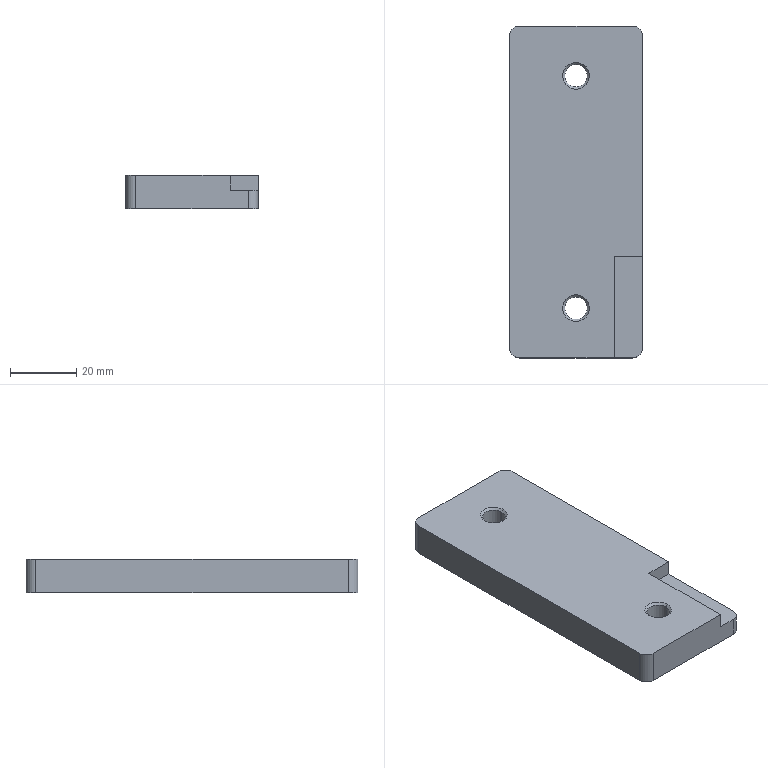Component | SolidWorks | FrameAssembly-1_FrameWeldment-1_MountingPlate-3 | 1 solid | 21 faces | box 40 x 100 x 10 mm | volume 38030 mm3 | plane 9 | cylinder 8 | cone 4 | commonest cylinder face diameters 6.8 x4 6 x4
build123d program:
from build123d import *

# Parameters (mm, degrees)
SKETCH1_2_W                = 40
SKETCH1_2_H                = 100
BOSS_EXTRUDE1_DEPTH        = 10
F_6_8_6_8_DIAMETER_HOLE1_D = 6.8
CHAMFER1_SIZE              = 0.625
FILLET1_R                  = 3
SKETCH1_W                  = 9
SKETCH1_H                  = 31
HOOK_CLEARANCE_SLOT_DEPTH  = 4.5


with BuildPart() as part:
    # Sketch1_2 → Boss-Extrude1 (new body)
    with BuildSketch(Plane.XY.offset(5)):
        Rectangle(SKETCH1_2_W, SKETCH1_2_H)
    extrude(amount=-BOSS_EXTRUDE1_DEPTH)

    # 6.8 _6.8_ Diameter Hole1 (through all)
    with Locations(Plane.XY.offset(5)):
        with Locations((0, -35), (0, 35)):
            Hole(F_6_8_6_8_DIAMETER_HOLE1_D / 2)

    # Chamfer1
    chamfer1_edges = [part.edges().sort_by_distance(p)[0] for p in [
        (3.4, 35, 5),
        (3.4, -35, 5),
    ]]
    chamfer(chamfer1_edges, length=CHAMFER1_SIZE)

    # Fillet1
    fillet1_edges = [part.edges().sort_by_distance(p)[0] for p in [
        (-20, -50, 0),
        (-20, 50, 0),
        (20, 50, 0),
        (20, -50, 0),
    ]]
    fillet(fillet1_edges, radius=FILLET1_R)

    # Sketch1 → Hook Clearance Slot (cut)
    with BuildSketch(Plane.XY.offset(5)):
        with Locations((16, -35)):
            Rectangle(SKETCH1_W, SKETCH1_H)
    extrude(amount=-HOOK_CLEARANCE_SLOT_DEPTH, mode=Mode.SUBTRACT)


solid = part.part

# Placed as in the assembly
solid = solid.moved(Location((43.754, -329.627, -371.5), (0, 0, 0)))
STEP:
#1=COLOUR_RGB('',0.7922,0.8196,0.9333);
#2=FILL_AREA_STYLE_COLOUR('',#1);
#3=FILL_AREA_STYLE('',(#2));
#4=SURFACE_STYLE_FILL_AREA(#3);
#5=SURFACE_SIDE_STYLE('',(#4));
#6=SURFACE_STYLE_USAGE(.BOTH.,#5);
#7=PRESENTATION_STYLE_ASSIGNMENT((#6));
#8=CARTESIAN_POINT('',(1.589,-14.355,-14.454));
#9=VERTEX_POINT('',#8);
#10=CARTESIAN_POINT('',(1.856,-14.355,-14.454));
#11=VERTEX_POINT('',#10);
#12=CARTESIAN_POINT('',(1.723,-14.355,-14.454));
#13=DIRECTION('',(0.,0.,1.));
#14=DIRECTION('',(1.,0.,0.));
#15=AXIS2_PLACEMENT_3D('',#12,#13,#14);
#16=CIRCLE('',#15,0.1339);
#17=EDGE_CURVE('',#9,#11,#16,.T.);
#18=ORIENTED_EDGE('',*,*,#17,.F.);
#19=CARTESIAN_POINT('',(1.564,-14.355,-14.429));
#20=VERTEX_POINT('',#19);
#21=CARTESIAN_POINT('',(1.589,-14.355,-14.454));
#22=DIRECTION('',(-0.7071,0.,0.7071));
#23=VECTOR('',#22,39.37);
#24=LINE('',#21,#23);
#25=EDGE_CURVE('',#9,#20,#24,.T.);
#26=ORIENTED_EDGE('',*,*,#25,.T.);
#27=CARTESIAN_POINT('',(1.881,-14.355,-14.429));
#28=VERTEX_POINT('',#27);
#29=CARTESIAN_POINT('',(1.723,-14.355,-14.429));
#30=DIRECTION('',(0.,0.,-1.));
#31=DIRECTION('',(1.,0.,0.));
#32=AXIS2_PLACEMENT_3D('',#29,#30,#31);
#33=CIRCLE('',#32,0.1585);
#34=EDGE_CURVE('',#28,#20,#33,.T.);
#35=ORIENTED_EDGE('',*,*,#34,.F.);
#36=CARTESIAN_POINT('',(1.856,-14.355,-14.454));
#37=DIRECTION('',(0.7071,0.,0.7071));
#38=VECTOR('',#37,39.37);
#39=LINE('',#36,#38);
#40=EDGE_CURVE('',#11,#28,#39,.T.);
#41=ORIENTED_EDGE('',*,*,#40,.F.);
#42=EDGE_LOOP('',(#18,#26,#35,#41));
#43=FACE_OUTER_BOUND('',#42,.T.);
#44=CARTESIAN_POINT('',(1.723,-14.355,-14.454));
#45=DIRECTION('',(0.,0.,1.));
#46=DIRECTION('',(1.,0.,0.));
#47=AXIS2_PLACEMENT_3D('',#44,#45,#46);
#48=CONICAL_SURFACE('',#47,0.1339,0.7854);
#49=ADVANCED_FACE('',(#43),#48,.F.);
#50=CARTESIAN_POINT('',(1.589,-11.599,-14.454));
#51=VERTEX_POINT('',#50);
#52=CARTESIAN_POINT('',(1.856,-11.599,-14.454));
#53=VERTEX_POINT('',#52);
#54=CARTESIAN_POINT('',(1.723,-11.599,-14.454));
#55=DIRECTION('',(0.,0.,1.));
#56=DIRECTION('',(1.,0.,0.));
#57=AXIS2_PLACEMENT_3D('',#54,#55,#56);
#58=CIRCLE('',#57,0.1339);
#59=EDGE_CURVE('',#51,#53,#58,.T.);
#60=ORIENTED_EDGE('',*,*,#59,.F.);
#61=CARTESIAN_POINT('',(1.564,-11.599,-14.429));
#62=VERTEX_POINT('',#61);
#63=CARTESIAN_POINT('',(1.589,-11.599,-14.454));
#64=DIRECTION('',(-0.7071,0.,0.7071));
#65=VECTOR('',#64,39.37);
#66=LINE('',#63,#65);
#67=EDGE_CURVE('',#51,#62,#66,.T.);
#68=ORIENTED_EDGE('',*,*,#67,.T.);
#69=CARTESIAN_POINT('',(1.881,-11.599,-14.429));
#70=VERTEX_POINT('',#69);
#71=CARTESIAN_POINT('',(1.723,-11.599,-14.429));
#72=DIRECTION('',(0.,0.,-1.));
#73=DIRECTION('',(1.,0.,0.));
#74=AXIS2_PLACEMENT_3D('',#71,#72,#73);
#75=CIRCLE('',#74,0.1585);
#76=EDGE_CURVE('',#70,#62,#75,.T.);
#77=ORIENTED_EDGE('',*,*,#76,.F.);
#78=CARTESIAN_POINT('',(1.856,-11.599,-14.454));
#79=DIRECTION('',(0.7071,0.,0.7071));
#80=VECTOR('',#79,39.37);
#81=LINE('',#78,#80);
#82=EDGE_CURVE('',#53,#70,#81,.T.);
#83=ORIENTED_EDGE('',*,*,#82,.F.);
#84=EDGE_LOOP('',(#60,#68,#77,#83));
#85=FACE_OUTER_BOUND('',#84,.T.);
#86=CARTESIAN_POINT('',(1.723,-11.599,-14.454));
#87=DIRECTION('',(0.,0.,1.));
#88=DIRECTION('',(1.,0.,0.));
#89=AXIS2_PLACEMENT_3D('',#86,#87,#88);
#90=CONICAL_SURFACE('',#89,0.1339,0.7854);
#91=ADVANCED_FACE('',(#85),#90,.F.);
#92=CARTESIAN_POINT('',(1.589,-14.355,-14.823));
#93=VERTEX_POINT('',#92);
#94=CARTESIAN_POINT('',(1.856,-14.355,-14.823));
#95=VERTEX_POINT('',#94);
#96=CARTESIAN_POINT('',(1.723,-14.355,-14.823));
#97=DIRECTION('',(0.,0.,1.));
#98=DIRECTION('',(1.,0.,0.));
#99=AXIS2_PLACEMENT_3D('',#96,#97,#98);
#100=CIRCLE('',#99,0.1339);
#101=EDGE_CURVE('',#93,#95,#100,.T.);
#102=ORIENTED_EDGE('',*,*,#101,.F.);
#103=CARTESIAN_POINT('',(1.589,-14.355,-14.429));
#104=DIRECTION('',(0.,0.,1.));
#105=VECTOR('',#104,39.37);
#106=LINE('',#103,#105);
#107=EDGE_CURVE('',#93,#9,#106,.T.);
#108=ORIENTED_EDGE('',*,*,#107,.T.);
#109=ORIENTED_EDGE('',*,*,#17,.T.);
#110=CARTESIAN_POINT('',(1.856,-14.355,-14.429));
#111=DIRECTION('',(0.,0.,1.));
#112=VECTOR('',#111,39.37);
#113=LINE('',#110,#112);
#114=EDGE_CURVE('',#95,#11,#113,.T.);
#115=ORIENTED_EDGE('',*,*,#114,.F.);
#116=EDGE_LOOP('',(#102,#108,#109,#115));
#117=FACE_OUTER_BOUND('',#116,.T.);
#118=CARTESIAN_POINT('',(1.723,-14.355,-14.429));
#119=DIRECTION('',(0.,0.,1.));
#120=DIRECTION('',(1.,0.,0.));
#121=AXIS2_PLACEMENT_3D('',#118,#119,#120);
#122=CYLINDRICAL_SURFACE('',#121,0.1339);
#123=ADVANCED_FACE('',(#117),#122,.F.);
#124=CARTESIAN_POINT('',(1.589,-11.599,-14.823));
#125=VERTEX_POINT('',#124);
#126=CARTESIAN_POINT('',(1.856,-11.599,-14.823));
#127=VERTEX_POINT('',#126);
#128=CARTESIAN_POINT('',(1.723,-11.599,-14.823));
#129=DIRECTION('',(0.,0.,1.));
#130=DIRECTION('',(1.,0.,0.));
#131=AXIS2_PLACEMENT_3D('',#128,#129,#130);
#132=CIRCLE('',#131,0.1339);
#133=EDGE_CURVE('',#125,#127,#132,.T.);
#134=ORIENTED_EDGE('',*,*,#133,.F.);
#135=CARTESIAN_POINT('',(1.589,-11.599,-14.429));
#136=DIRECTION('',(0.,0.,1.));
#137=VECTOR('',#136,39.37);
#138=LINE('',#135,#137);
#139=EDGE_CURVE('',#125,#51,#138,.T.);
#140=ORIENTED_EDGE('',*,*,#139,.T.);
#141=ORIENTED_EDGE('',*,*,#59,.T.);
#142=CARTESIAN_POINT('',(1.856,-11.599,-14.429));
#143=DIRECTION('',(0.,0.,1.));
#144=VECTOR('',#143,39.37);
#145=LINE('',#142,#144);
#146=EDGE_CURVE('',#127,#53,#145,.T.);
#147=ORIENTED_EDGE('',*,*,#146,.F.);
#148=EDGE_LOOP('',(#134,#140,#141,#147));
#149=FACE_OUTER_BOUND('',#148,.T.);
#150=CARTESIAN_POINT('',(1.723,-11.599,-14.429));
#151=DIRECTION('',(0.,0.,1.));
#152=DIRECTION('',(1.,0.,0.));
#153=AXIS2_PLACEMENT_3D('',#150,#151,#152);
#154=CYLINDRICAL_SURFACE('',#153,0.1339);
#155=ADVANCED_FACE('',(#149),#154,.F.);
#156=CARTESIAN_POINT('',(2.51,-14.828,-14.606));
#157=VERTEX_POINT('',#156);
#158=CARTESIAN_POINT('',(2.51,-14.828,-14.823));
#159=VERTEX_POINT('',#158);
#160=CARTESIAN_POINT('',(2.51,-14.828,-14.823));
#161=DIRECTION('',(0.,0.,-1.));
#162=VECTOR('',#161,39.37);
#163=LINE('',#160,#162);
#164=EDGE_CURVE('',#157,#159,#163,.T.);
#165=ORIENTED_EDGE('',*,*,#164,.F.);
#166=CARTESIAN_POINT('',(2.392,-14.946,-14.606));
#167=VERTEX_POINT('',#166);
#168=CARTESIAN_POINT('',(2.392,-14.828,-14.606));
#169=DIRECTION('',(0.,0.,-1.));
#170=DIRECTION('',(1.,0.,0.));
#171=AXIS2_PLACEMENT_3D('',#168,#169,#170);
#172=CIRCLE('',#171,0.1181);
#173=EDGE_CURVE('',#157,#167,#172,.T.);
#174=ORIENTED_EDGE('',*,*,#173,.T.);
#175=CARTESIAN_POINT('',(2.392,-14.946,-14.823));
#176=VERTEX_POINT('',#175);
#177=CARTESIAN_POINT('',(2.392,-14.946,-14.823));
#178=DIRECTION('',(0.,0.,1.));
#179=VECTOR('',#178,39.37);
#180=LINE('',#177,#179);
#181=EDGE_CURVE('',#176,#167,#180,.T.);
#182=ORIENTED_EDGE('',*,*,#181,.F.);
#183=CARTESIAN_POINT('',(2.392,-14.828,-14.823));
#184=DIRECTION('',(0.,0.,-1.));
#185=DIRECTION('',(1.,0.,0.));
#186=AXIS2_PLACEMENT_3D('',#183,#184,#185);
#187=CIRCLE('',#186,0.1181);
#188=EDGE_CURVE('',#159,#176,#187,.T.);
#189=ORIENTED_EDGE('',*,*,#188,.F.);
#190=EDGE_LOOP('',(#165,#174,#182,#189));
#191=FACE_OUTER_BOUND('',#190,.T.);
#192=CARTESIAN_POINT('',(2.392,-14.828,-14.823));
#193=DIRECTION('',(0.,0.,1.));
#194=DIRECTION('',(1.,0.,0.));
#195=AXIS2_PLACEMENT_3D('',#192,#193,#194);
#196=CYLINDRICAL_SURFACE('',#195,0.1181);
#197=ADVANCED_FACE('',(#191),#196,.T.);
#198=CARTESIAN_POINT('',(2.175,-14.946,-14.429));
#199=VERTEX_POINT('',#198);
#200=CARTESIAN_POINT('',(2.175,-14.946,-14.606));
#201=VERTEX_POINT('',#200);
#202=CARTESIAN_POINT('',(2.175,-14.946,-14.823));
#203=DIRECTION('',(0.,0.,-1.));
#204=VECTOR('',#203,39.37);
#205=LINE('',#202,#204);
#206=EDGE_CURVE('',#199,#201,#205,.T.);
#207=ORIENTED_EDGE('',*,*,#206,.F.);
#208=CARTESIAN_POINT('',(1.053,-14.946,-14.429));
#209=VERTEX_POINT('',#208);
#210=CARTESIAN_POINT('',(0.9352,-14.946,-14.429));
#211=DIRECTION('',(1.,0.,0.));
#212=VECTOR('',#211,39.37);
#213=LINE('',#210,#212);
#214=EDGE_CURVE('',#209,#199,#213,.T.);
#215=ORIENTED_EDGE('',*,*,#214,.F.);
#216=CARTESIAN_POINT('',(1.053,-14.946,-14.823));
#217=VERTEX_POINT('',#216);
#218=CARTESIAN_POINT('',(1.053,-14.946,-14.823));
#219=DIRECTION('',(0.,0.,-1.));
#220=VECTOR('',#219,39.37);
#221=LINE('',#218,#220);
#222=EDGE_CURVE('',#209,#217,#221,.T.);
#223=ORIENTED_EDGE('',*,*,#222,.T.);
#224=CARTESIAN_POINT('',(0.9352,-14.946,-14.823));
#225=DIRECTION('',(1.,0.,0.));
#226=VECTOR('',#225,39.37);
#227=LINE('',#224,#226);
#228=EDGE_CURVE('',#217,#176,#227,.T.);
#229=ORIENTED_EDGE('',*,*,#228,.T.);
#230=ORIENTED_EDGE('',*,*,#181,.T.);
#231=CARTESIAN_POINT('',(0.9352,-14.946,-14.606));
#232=DIRECTION('',(-1.,0.,0.));
#233=VECTOR('',#232,39.37);
#234=LINE('',#231,#233);
#235=EDGE_CURVE('',#167,#201,#234,.T.);
#236=ORIENTED_EDGE('',*,*,#235,.T.);
#237=EDGE_LOOP('',(#207,#215,#223,#229,#230,#236));
#238=FACE_OUTER_BOUND('',#237,.T.);
#239=CARTESIAN_POINT('',(0.9352,-14.946,-14.823));
#240=DIRECTION('',(0.,-1.,0.));
#241=DIRECTION('',(0.,0.,-1.));
#242=AXIS2_PLACEMENT_3D('',#239,#240,#241);
#243=PLANE('',#242);
#244=ADVANCED_FACE('',(#238),#243,.T.);
#245=CARTESIAN_POINT('',(0.9352,-11.127,-14.429));
#246=VERTEX_POINT('',#245);
#247=CARTESIAN_POINT('',(0.9352,-14.828,-14.429));
#248=VERTEX_POINT('',#247);
#249=CARTESIAN_POINT('',(0.9352,-11.009,-14.429));
#250=DIRECTION('',(0.,-1.,0.));
#251=VECTOR('',#250,39.37);
#252=LINE('',#249,#251);
#253=EDGE_CURVE('',#246,#248,#252,.T.);
#254=ORIENTED_EDGE('',*,*,#253,.F.);
#255=CARTESIAN_POINT('',(0.9352,-11.127,-14.823));
#256=VERTEX_POINT('',#255);
#257=CARTESIAN_POINT('',(0.9352,-11.127,-14.823));
#258=DIRECTION('',(0.,0.,-1.));
#259=VECTOR('',#258,39.37);
#260=LINE('',#257,#259);
#261=EDGE_CURVE('',#246,#256,#260,.T.);
#262=ORIENTED_EDGE('',*,*,#261,.T.);
#263=CARTESIAN_POINT('',(0.9352,-14.828,-14.823));
#264=VERTEX_POINT('',#263);
#265=CARTESIAN_POINT('',(0.9352,-11.009,-14.823));
#266=DIRECTION('',(0.,-1.,0.));
#267=VECTOR('',#266,39.37);
#268=LINE('',#265,#267);
#269=EDGE_CURVE('',#256,#264,#268,.T.);
#270=ORIENTED_EDGE('',*,*,#269,.T.);
#271=CARTESIAN_POINT('',(0.9352,-14.828,-14.823));
#272=DIRECTION('',(0.,0.,1.));
#273=VECTOR('',#272,39.37);
#274=LINE('',#271,#273);
#275=EDGE_CURVE('',#264,#248,#274,.T.);
#276=ORIENTED_EDGE('',*,*,#275,.T.);
#277=EDGE_LOOP('',(#254,#262,#270,#276));
#278=FACE_OUTER_BOUND('',#277,.T.);
#279=CARTESIAN_POINT('',(0.9352,-11.009,-14.823));
#280=DIRECTION('',(-1.,-0.,0.));
#281=DIRECTION('',(0.,-1.,0.));
#282=AXIS2_PLACEMENT_3D('',#279,#280,#281);
#283=PLANE('',#282);
#284=ADVANCED_FACE('',(#278),#283,.T.);
#285=CARTESIAN_POINT('',(2.392,-11.009,-14.823));
#286=VERTEX_POINT('',#285);
#287=CARTESIAN_POINT('',(1.053,-11.009,-14.823));
#288=VERTEX_POINT('',#287);
#289=CARTESIAN_POINT('',(2.51,-11.009,-14.823));
#290=DIRECTION('',(-1.,0.,0.));
#291=VECTOR('',#290,39.37);
#292=LINE('',#289,#291);
#293=EDGE_CURVE('',#286,#288,#292,.T.);
#294=ORIENTED_EDGE('',*,*,#293,.T.);
#295=CARTESIAN_POINT('',(1.053,-11.009,-14.429));
#296=VERTEX_POINT('',#295);
#297=CARTESIAN_POINT('',(1.053,-11.009,-14.823));
#298=DIRECTION('',(0.,0.,1.));
#299=VECTOR('',#298,39.37);
#300=LINE('',#297,#299);
#301=EDGE_CURVE('',#288,#296,#300,.T.);
#302=ORIENTED_EDGE('',*,*,#301,.T.);
#303=CARTESIAN_POINT('',(2.392,-11.009,-14.429));
#304=VERTEX_POINT('',#303);
#305=CARTESIAN_POINT('',(2.51,-11.009,-14.429));
#306=DIRECTION('',(-1.,0.,0.));
#307=VECTOR('',#306,39.37);
#308=LINE('',#305,#307);
#309=EDGE_CURVE('',#304,#296,#308,.T.);
#310=ORIENTED_EDGE('',*,*,#309,.F.);
#311=CARTESIAN_POINT('',(2.392,-11.009,-14.823));
#312=DIRECTION('',(0.,0.,-1.));
#313=VECTOR('',#312,39.37);
#314=LINE('',#311,#313);
#315=EDGE_CURVE('',#304,#286,#314,.T.);
#316=ORIENTED_EDGE('',*,*,#315,.T.);
#317=EDGE_LOOP('',(#294,#302,#310,#316));
#318=FACE_OUTER_BOUND('',#317,.T.);
#319=CARTESIAN_POINT('',(2.51,-11.009,-14.823));
#320=DIRECTION('',(0.,1.,0.));
#321=DIRECTION('',(0.,0.,1.));
#322=AXIS2_PLACEMENT_3D('',#319,#320,#321);
#323=PLANE('',#322);
#324=ADVANCED_FACE('',(#318),#323,.T.);
#325=CARTESIAN_POINT('',(2.51,-13.745,-14.606));
#326=VERTEX_POINT('',#325);
#327=CARTESIAN_POINT('',(2.51,-13.745,-14.429));
#328=VERTEX_POINT('',#327);
#329=CARTESIAN_POINT('',(2.51,-13.745,-14.823));
#330=DIRECTION('',(0.,0.,1.));
#331=VECTOR('',#330,39.37);
#332=LINE('',#329,#331);
#333=EDGE_CURVE('',#326,#328,#332,.T.);
#334=ORIENTED_EDGE('',*,*,#333,.F.);
#335=CARTESIAN_POINT('',(2.51,-14.946,-14.606));
#336=DIRECTION('',(0.,-1.,0.));
#337=VECTOR('',#336,39.37);
#338=LINE('',#335,#337);
#339=EDGE_CURVE('',#326,#157,#338,.T.);
#340=ORIENTED_EDGE('',*,*,#339,.T.);
#341=ORIENTED_EDGE('',*,*,#164,.T.);
#342=CARTESIAN_POINT('',(2.51,-11.127,-14.823));
#343=VERTEX_POINT('',#342);
#344=CARTESIAN_POINT('',(2.51,-14.946,-14.823));
#345=DIRECTION('',(-0.,1.,0.));
#346=VECTOR('',#345,39.37);
#347=LINE('',#344,#346);
#348=EDGE_CURVE('',#159,#343,#347,.T.);
#349=ORIENTED_EDGE('',*,*,#348,.T.);
#350=CARTESIAN_POINT('',(2.51,-11.127,-14.429));
#351=VERTEX_POINT('',#350);
#352=CARTESIAN_POINT('',(2.51,-11.127,-14.823));
#353=DIRECTION('',(0.,0.,1.));
#354=VECTOR('',#353,39.37);
#355=LINE('',#352,#354);
#356=EDGE_CURVE('',#343,#351,#355,.T.);
#357=ORIENTED_EDGE('',*,*,#356,.T.);
#358=CARTESIAN_POINT('',(2.51,-14.946,-14.429));
#359=DIRECTION('',(-0.,1.,0.));
#360=VECTOR('',#359,39.37);
#361=LINE('',#358,#360);
#362=EDGE_CURVE('',#328,#351,#361,.T.);
#363=ORIENTED_EDGE('',*,*,#362,.F.);
#364=EDGE_LOOP('',(#334,#340,#341,#349,#357,#363));
#365=FACE_OUTER_BOUND('',#364,.T.);
#366=CARTESIAN_POINT('',(2.51,-14.946,-14.823));
#367=DIRECTION('',(1.,0.,0.));
#368=DIRECTION('',(-0.,1.,0.));
#369=AXIS2_PLACEMENT_3D('',#366,#367,#368);
#370=PLANE('',#369);
#371=ADVANCED_FACE('',(#365),#370,.T.);
#372=CARTESIAN_POINT('',(1.723,-14.355,-14.823));
#373=DIRECTION('',(0.,0.,1.));
#374=DIRECTION('',(1.,0.,0.));
#375=AXIS2_PLACEMENT_3D('',#372,#373,#374);
#376=CIRCLE('',#375,0.1339);
#377=EDGE_CURVE('',#95,#93,#376,.T.);
#378=ORIENTED_EDGE('',*,*,#377,.T.);
#379=ORIENTED_EDGE('',*,*,#101,.T.);
#380=EDGE_LOOP('',(#378,#379));
#381=FACE_BOUND('',#380,.T.);
#382=CARTESIAN_POINT('',(1.723,-11.599,-14.823));
#383=DIRECTION('',(0.,0.,1.));
#384=DIRECTION('',(1.,0.,0.));
#385=AXIS2_PLACEMENT_3D('',#382,#383,#384);
#386=CIRCLE('',#385,0.1339);
#387=EDGE_CURVE('',#127,#125,#386,.T.);
#388=ORIENTED_EDGE('',*,*,#387,.T.);
#389=ORIENTED_EDGE('',*,*,#133,.T.);
#390=EDGE_LOOP('',(#388,#389));
#391=FACE_BOUND('',#390,.T.);
#392=ORIENTED_EDGE('',*,*,#269,.F.);
#393=CARTESIAN_POINT('',(1.053,-11.127,-14.823));
#394=DIRECTION('',(0.,0.,-1.));
#395=DIRECTION('',(1.,0.,0.));
#396=AXIS2_PLACEMENT_3D('',#393,#394,#395);
#397=CIRCLE('',#396,0.1181);
#398=EDGE_CURVE('',#256,#288,#397,.T.);
#399=ORIENTED_EDGE('',*,*,#398,.T.);
#400=ORIENTED_EDGE('',*,*,#293,.F.);
#401=CARTESIAN_POINT('',(2.392,-11.127,-14.823));
#402=DIRECTION('',(0.,0.,-1.));
#403=DIRECTION('',(1.,0.,0.));
#404=AXIS2_PLACEMENT_3D('',#401,#402,#403);
#405=CIRCLE('',#404,0.1181);
#406=EDGE_CURVE('',#286,#343,#405,.T.);
#407=ORIENTED_EDGE('',*,*,#406,.T.);
#408=ORIENTED_EDGE('',*,*,#348,.F.);
#409=ORIENTED_EDGE('',*,*,#188,.T.);
#410=ORIENTED_EDGE('',*,*,#228,.F.);
#411=CARTESIAN_POINT('',(1.053,-14.828,-14.823));
#412=DIRECTION('',(0.,0.,-1.));
#413=DIRECTION('',(1.,0.,0.));
#414=AXIS2_PLACEMENT_3D('',#411,#412,#413);
#415=CIRCLE('',#414,0.1181);
#416=EDGE_CURVE('',#217,#264,#415,.T.);
#417=ORIENTED_EDGE('',*,*,#416,.T.);
#418=EDGE_LOOP('',(#392,#399,#400,#407,#408,#409,#410,#417));
#419=FACE_OUTER_BOUND('',#418,.T.);
#420=CARTESIAN_POINT('',(1.723,-12.977,-14.823));
#421=DIRECTION('',(0.,0.,1.));
#422=DIRECTION('',(1.,0.,0.));
#423=AXIS2_PLACEMENT_3D('',#420,#421,#422);
#424=PLANE('',#423);
#425=ADVANCED_FACE('',(#381,#391,#419),#424,.F.);
#426=CARTESIAN_POINT('',(2.175,-13.745,-14.429));
#427=VERTEX_POINT('',#426);
#428=CARTESIAN_POINT('',(2.175,-13.745,-14.429));
#429=DIRECTION('',(0.,-1.,0.));
#430=VECTOR('',#429,39.37);
#431=LINE('',#428,#430);
#432=EDGE_CURVE('',#427,#199,#431,.T.);
#433=ORIENTED_EDGE('',*,*,#432,.F.);
#434=CARTESIAN_POINT('',(2.53,-13.745,-14.429));
#435=DIRECTION('',(-1.,0.,0.));
#436=VECTOR('',#435,39.37);
#437=LINE('',#434,#436);
#438=EDGE_CURVE('',#328,#427,#437,.T.);
#439=ORIENTED_EDGE('',*,*,#438,.F.);
#440=ORIENTED_EDGE('',*,*,#362,.T.);
#441=CARTESIAN_POINT('',(2.392,-11.127,-14.429));
#442=DIRECTION('',(0.,0.,1.));
#443=DIRECTION('',(1.,0.,0.));
#444=AXIS2_PLACEMENT_3D('',#441,#442,#443);
#445=CIRCLE('',#444,0.1181);
#446=EDGE_CURVE('',#351,#304,#445,.T.);
#447=ORIENTED_EDGE('',*,*,#446,.T.);
#448=ORIENTED_EDGE('',*,*,#309,.T.);
#449=CARTESIAN_POINT('',(1.053,-11.127,-14.429));
#450=DIRECTION('',(0.,0.,1.));
#451=DIRECTION('',(1.,0.,0.));
#452=AXIS2_PLACEMENT_3D('',#449,#450,#451);
#453=CIRCLE('',#452,0.1181);
#454=EDGE_CURVE('',#296,#246,#453,.T.);
#455=ORIENTED_EDGE('',*,*,#454,.T.);
#456=ORIENTED_EDGE('',*,*,#253,.T.);
#457=CARTESIAN_POINT('',(1.053,-14.828,-14.429));
#458=DIRECTION('',(0.,0.,1.));
#459=DIRECTION('',(1.,0.,0.));
#460=AXIS2_PLACEMENT_3D('',#457,#458,#459);
#461=CIRCLE('',#460,0.1181);
#462=EDGE_CURVE('',#248,#209,#461,.T.);
#463=ORIENTED_EDGE('',*,*,#462,.T.);
#464=ORIENTED_EDGE('',*,*,#214,.T.);
#465=EDGE_LOOP('',(#433,#439,#440,#447,#448,#455,#456,#463,#464));
#466=FACE_OUTER_BOUND('',#465,.T.);
#467=ORIENTED_EDGE('',*,*,#76,.T.);
#468=CARTESIAN_POINT('',(1.723,-11.599,-14.429));
#469=DIRECTION('',(0.,0.,-1.));
#470=DIRECTION('',(1.,0.,0.));
#471=AXIS2_PLACEMENT_3D('',#468,#469,#470);
#472=CIRCLE('',#471,0.1585);
#473=EDGE_CURVE('',#62,#70,#472,.T.);
#474=ORIENTED_EDGE('',*,*,#473,.T.);
#475=EDGE_LOOP('',(#467,#474));
#476=FACE_BOUND('',#475,.T.);
#477=ORIENTED_EDGE('',*,*,#34,.T.);
#478=CARTESIAN_POINT('',(1.723,-14.355,-14.429));
#479=DIRECTION('',(0.,0.,-1.));
#480=DIRECTION('',(1.,0.,0.));
#481=AXIS2_PLACEMENT_3D('',#478,#479,#480);
#482=CIRCLE('',#481,0.1585);
#483=EDGE_CURVE('',#20,#28,#482,.T.);
#484=ORIENTED_EDGE('',*,*,#483,.T.);
#485=EDGE_LOOP('',(#477,#484));
#486=FACE_BOUND('',#485,.T.);
#487=CARTESIAN_POINT('',(1.723,-12.977,-14.429));
#488=DIRECTION('',(0.,0.,1.));
#489=DIRECTION('',(1.,0.,0.));
#490=AXIS2_PLACEMENT_3D('',#487,#488,#489);
#491=PLANE('',#490);
#492=ADVANCED_FACE('',(#466,#476,#486),#491,.T.);
#493=ORIENTED_EDGE('',*,*,#139,.F.);
#494=ORIENTED_EDGE('',*,*,#387,.F.);
#495=ORIENTED_EDGE('',*,*,#146,.T.);
#496=CARTESIAN_POINT('',(1.723,-11.599,-14.454));
#497=DIRECTION('',(0.,0.,1.));
#498=DIRECTION('',(1.,0.,0.));
#499=AXIS2_PLACEMENT_3D('',#496,#497,#498);
#500=CIRCLE('',#499,0.1339);
#501=EDGE_CURVE('',#53,#51,#500,.T.);
#502=ORIENTED_EDGE('',*,*,#501,.T.);
#503=EDGE_LOOP('',(#493,#494,#495,#502));
#504=FACE_OUTER_BOUND('',#503,.T.);
#505=CARTESIAN_POINT('',(1.723,-11.599,-14.429));
#506=DIRECTION('',(0.,0.,1.));
#507=DIRECTION('',(1.,0.,0.));
#508=AXIS2_PLACEMENT_3D('',#505,#506,#507);
#509=CYLINDRICAL_SURFACE('',#508,0.1339);
#510=ADVANCED_FACE('',(#504),#509,.F.);
#511=ORIENTED_EDGE('',*,*,#107,.F.);
#512=ORIENTED_EDGE('',*,*,#377,.F.);
#513=ORIENTED_EDGE('',*,*,#114,.T.);
#514=CARTESIAN_POINT('',(1.723,-14.355,-14.454));
#515=DIRECTION('',(0.,0.,1.));
#516=DIRECTION('',(1.,0.,0.));
#517=AXIS2_PLACEMENT_3D('',#514,#515,#516);
#518=CIRCLE('',#517,0.1339);
#519=EDGE_CURVE('',#11,#9,#518,.T.);
#520=ORIENTED_EDGE('',*,*,#519,.T.);
#521=EDGE_LOOP('',(#511,#512,#513,#520));
#522=FACE_OUTER_BOUND('',#521,.T.);
#523=CARTESIAN_POINT('',(1.723,-14.355,-14.429));
#524=DIRECTION('',(0.,0.,1.));
#525=DIRECTION('',(1.,0.,0.));
#526=AXIS2_PLACEMENT_3D('',#523,#524,#525);
#527=CYLINDRICAL_SURFACE('',#526,0.1339);
#528=ADVANCED_FACE('',(#522),#527,.F.);
#529=ORIENTED_EDGE('',*,*,#67,.F.);
#530=ORIENTED_EDGE('',*,*,#501,.F.);
#531=ORIENTED_EDGE('',*,*,#82,.T.);
#532=ORIENTED_EDGE('',*,*,#473,.F.);
#533=EDGE_LOOP('',(#529,#530,#531,#532));
#534=FACE_OUTER_BOUND('',#533,.T.);
#535=CARTESIAN_POINT('',(1.723,-11.599,-14.454));
#536=DIRECTION('',(0.,0.,1.));
#537=DIRECTION('',(1.,0.,0.));
#538=AXIS2_PLACEMENT_3D('',#535,#536,#537);
#539=CONICAL_SURFACE('',#538,0.1339,0.7854);
#540=ADVANCED_FACE('',(#534),#539,.F.);
#541=ORIENTED_EDGE('',*,*,#25,.F.);
#542=ORIENTED_EDGE('',*,*,#519,.F.);
#543=ORIENTED_EDGE('',*,*,#40,.T.);
#544=ORIENTED_EDGE('',*,*,#483,.F.);
#545=EDGE_LOOP('',(#541,#542,#543,#544));
#546=FACE_OUTER_BOUND('',#545,.T.);
#547=CARTESIAN_POINT('',(1.723,-14.355,-14.454));
#548=DIRECTION('',(0.,0.,1.));
#549=DIRECTION('',(1.,0.,0.));
#550=AXIS2_PLACEMENT_3D('',#547,#548,#549);
#551=CONICAL_SURFACE('',#550,0.1339,0.7854);
#552=ADVANCED_FACE('',(#546),#551,.F.);
#553=ORIENTED_EDGE('',*,*,#398,.F.);
#554=ORIENTED_EDGE('',*,*,#261,.F.);
#555=ORIENTED_EDGE('',*,*,#454,.F.);
#556=ORIENTED_EDGE('',*,*,#301,.F.);
#557=EDGE_LOOP('',(#553,#554,#555,#556));
#558=FACE_OUTER_BOUND('',#557,.T.);
#559=CARTESIAN_POINT('',(1.053,-11.127,-14.823));
#560=DIRECTION('',(0.,0.,1.));
#561=DIRECTION('',(1.,0.,0.));
#562=AXIS2_PLACEMENT_3D('',#559,#560,#561);
#563=CYLINDRICAL_SURFACE('',#562,0.1181);
#564=ADVANCED_FACE('',(#558),#563,.T.);
#565=ORIENTED_EDGE('',*,*,#406,.F.);
#566=ORIENTED_EDGE('',*,*,#315,.F.);
#567=ORIENTED_EDGE('',*,*,#446,.F.);
#568=ORIENTED_EDGE('',*,*,#356,.F.);
#569=EDGE_LOOP('',(#565,#566,#567,#568));
#570=FACE_OUTER_BOUND('',#569,.T.);
#571=CARTESIAN_POINT('',(2.392,-11.127,-14.823));
#572=DIRECTION('',(0.,0.,1.));
#573=DIRECTION('',(1.,0.,0.));
#574=AXIS2_PLACEMENT_3D('',#571,#572,#573);
#575=CYLINDRICAL_SURFACE('',#574,0.1181);
#576=ADVANCED_FACE('',(#570),#575,.T.);
#577=ORIENTED_EDGE('',*,*,#416,.F.);
#578=ORIENTED_EDGE('',*,*,#222,.F.);
#579=ORIENTED_EDGE('',*,*,#462,.F.);
#580=ORIENTED_EDGE('',*,*,#275,.F.);
#581=EDGE_LOOP('',(#577,#578,#579,#580));
#582=FACE_OUTER_BOUND('',#581,.T.);
#583=CARTESIAN_POINT('',(1.053,-14.828,-14.823));
#584=DIRECTION('',(0.,0.,1.));
#585=DIRECTION('',(1.,0.,0.));
#586=AXIS2_PLACEMENT_3D('',#583,#584,#585);
#587=CYLINDRICAL_SURFACE('',#586,0.1181);
#588=ADVANCED_FACE('',(#582),#587,.T.);
#589=ORIENTED_EDGE('',*,*,#206,.T.);
#590=CARTESIAN_POINT('',(2.175,-13.745,-14.606));
#591=VERTEX_POINT('',#590);
#592=CARTESIAN_POINT('',(2.175,-13.745,-14.606));
#593=DIRECTION('',(0.,-1.,0.));
#594=VECTOR('',#593,39.37);
#595=LINE('',#592,#594);
#596=EDGE_CURVE('',#591,#201,#595,.T.);
#597=ORIENTED_EDGE('',*,*,#596,.F.);
#598=CARTESIAN_POINT('',(2.175,-13.745,-14.606));
#599=DIRECTION('',(0.,0.,1.));
#600=VECTOR('',#599,39.37);
#601=LINE('',#598,#600);
#602=EDGE_CURVE('',#591,#427,#601,.T.);
#603=ORIENTED_EDGE('',*,*,#602,.T.);
#604=ORIENTED_EDGE('',*,*,#432,.T.);
#605=EDGE_LOOP('',(#589,#597,#603,#604));
#606=FACE_OUTER_BOUND('',#605,.T.);
#607=CARTESIAN_POINT('',(2.175,-13.745,-14.606));
#608=DIRECTION('',(-1.,0.,0.));
#609=DIRECTION('',(0.,0.,1.));
#610=AXIS2_PLACEMENT_3D('',#607,#608,#609);
#611=PLANE('',#610);
#612=ADVANCED_FACE('',(#606),#611,.F.);
#613=ORIENTED_EDGE('',*,*,#333,.T.);
#614=ORIENTED_EDGE('',*,*,#438,.T.);
#615=ORIENTED_EDGE('',*,*,#602,.F.);
#616=CARTESIAN_POINT('',(2.53,-13.745,-14.606));
#617=DIRECTION('',(-1.,0.,0.));
#618=VECTOR('',#617,39.37);
#619=LINE('',#616,#618);
#620=EDGE_CURVE('',#326,#591,#619,.T.);
#621=ORIENTED_EDGE('',*,*,#620,.F.);
#622=EDGE_LOOP('',(#613,#614,#615,#621));
#623=FACE_OUTER_BOUND('',#622,.T.);
#624=CARTESIAN_POINT('',(2.53,-13.745,-14.606));
#625=DIRECTION('',(0.,1.,0.));
#626=DIRECTION('',(0.,0.,1.));
#627=AXIS2_PLACEMENT_3D('',#624,#625,#626);
#628=PLANE('',#627);
#629=ADVANCED_FACE('',(#623),#628,.F.);
#630=ORIENTED_EDGE('',*,*,#173,.F.);
#631=ORIENTED_EDGE('',*,*,#339,.F.);
#632=ORIENTED_EDGE('',*,*,#620,.T.);
#633=ORIENTED_EDGE('',*,*,#596,.T.);
#634=ORIENTED_EDGE('',*,*,#235,.F.);
#635=EDGE_LOOP('',(#630,#631,#632,#633,#634));
#636=FACE_OUTER_BOUND('',#635,.T.);
#637=CARTESIAN_POINT('',(1.723,-12.977,-14.606));
#638=DIRECTION('',(0.,0.,1.));
#639=DIRECTION('',(1.,0.,0.));
#640=AXIS2_PLACEMENT_3D('',#637,#638,#639);
#641=PLANE('',#640);
#642=ADVANCED_FACE('',(#636),#641,.T.);
#643=CLOSED_SHELL('',(#49,#91,#123,#155,#197,#244,#284,#324,#371,#425,#492,#510,#528,#540,#552,#564,#576,#588,#612,#629,#642));
#644=MANIFOLD_SOLID_BREP('',#643);
#645=STYLED_ITEM('',(#7),#644);
#646=(LENGTH_UNIT()NAMED_UNIT(*)SI_UNIT($,.METRE.));
#647=LENGTH_MEASURE_WITH_UNIT(LENGTH_MEASURE(0.0254),#646);
#648=DIMENSIONAL_EXPONENTS(1.,0.,0.,0.,0.,0.,0.);
#649=(CONVERSION_BASED_UNIT('',#647)LENGTH_UNIT()NAMED_UNIT(#648));
#650=UNCERTAINTY_MEASURE_WITH_UNIT(LENGTH_MEASURE(0.00001),#649,'','');
#651=(NAMED_UNIT(*)PLANE_ANGLE_UNIT()SI_UNIT($,.RADIAN.));
#652=(NAMED_UNIT(*)SI_UNIT($,.STERADIAN.)SOLID_ANGLE_UNIT());
#653=(GEOMETRIC_REPRESENTATION_CONTEXT(3)GLOBAL_UNCERTAINTY_ASSIGNED_CONTEXT((#650))GLOBAL_UNIT_ASSIGNED_CONTEXT((#649,#651,#652))REPRESENTATION_CONTEXT('',''));
#654=MECHANICAL_DESIGN_GEOMETRIC_PRESENTATION_REPRESENTATION('',(#645),#653);
#655=PRESENTATION_LAYER_ASSIGNMENT('','',(#645));
#656=CARTESIAN_POINT('',(0.,0.,0.));
#657=DIRECTION('',(0.,0.,1.));
#658=DIRECTION('',(1.,0.,0.));
#659=AXIS2_PLACEMENT_3D('',#656,#657,#658);
#660=(LENGTH_UNIT()NAMED_UNIT(*)SI_UNIT($,.METRE.));
#661=LENGTH_MEASURE_WITH_UNIT(LENGTH_MEASURE(0.0254),#660);
#662=DIMENSIONAL_EXPONENTS(1.,0.,0.,0.,0.,0.,0.);
#663=(CONVERSION_BASED_UNIT('',#661)LENGTH_UNIT()NAMED_UNIT(#662));
#664=UNCERTAINTY_MEASURE_WITH_UNIT(LENGTH_MEASURE(0.00001),#663,'','');
#665=(NAMED_UNIT(*)PLANE_ANGLE_UNIT()SI_UNIT($,.RADIAN.));
#666=(NAMED_UNIT(*)SI_UNIT($,.STERADIAN.)SOLID_ANGLE_UNIT());
#667=(GEOMETRIC_REPRESENTATION_CONTEXT(3)GLOBAL_UNCERTAINTY_ASSIGNED_CONTEXT((#664))GLOBAL_UNIT_ASSIGNED_CONTEXT((#663,#665,#666))REPRESENTATION_CONTEXT('',''));
#668=ADVANCED_BREP_SHAPE_REPRESENTATION('',(#644,#659),#667);